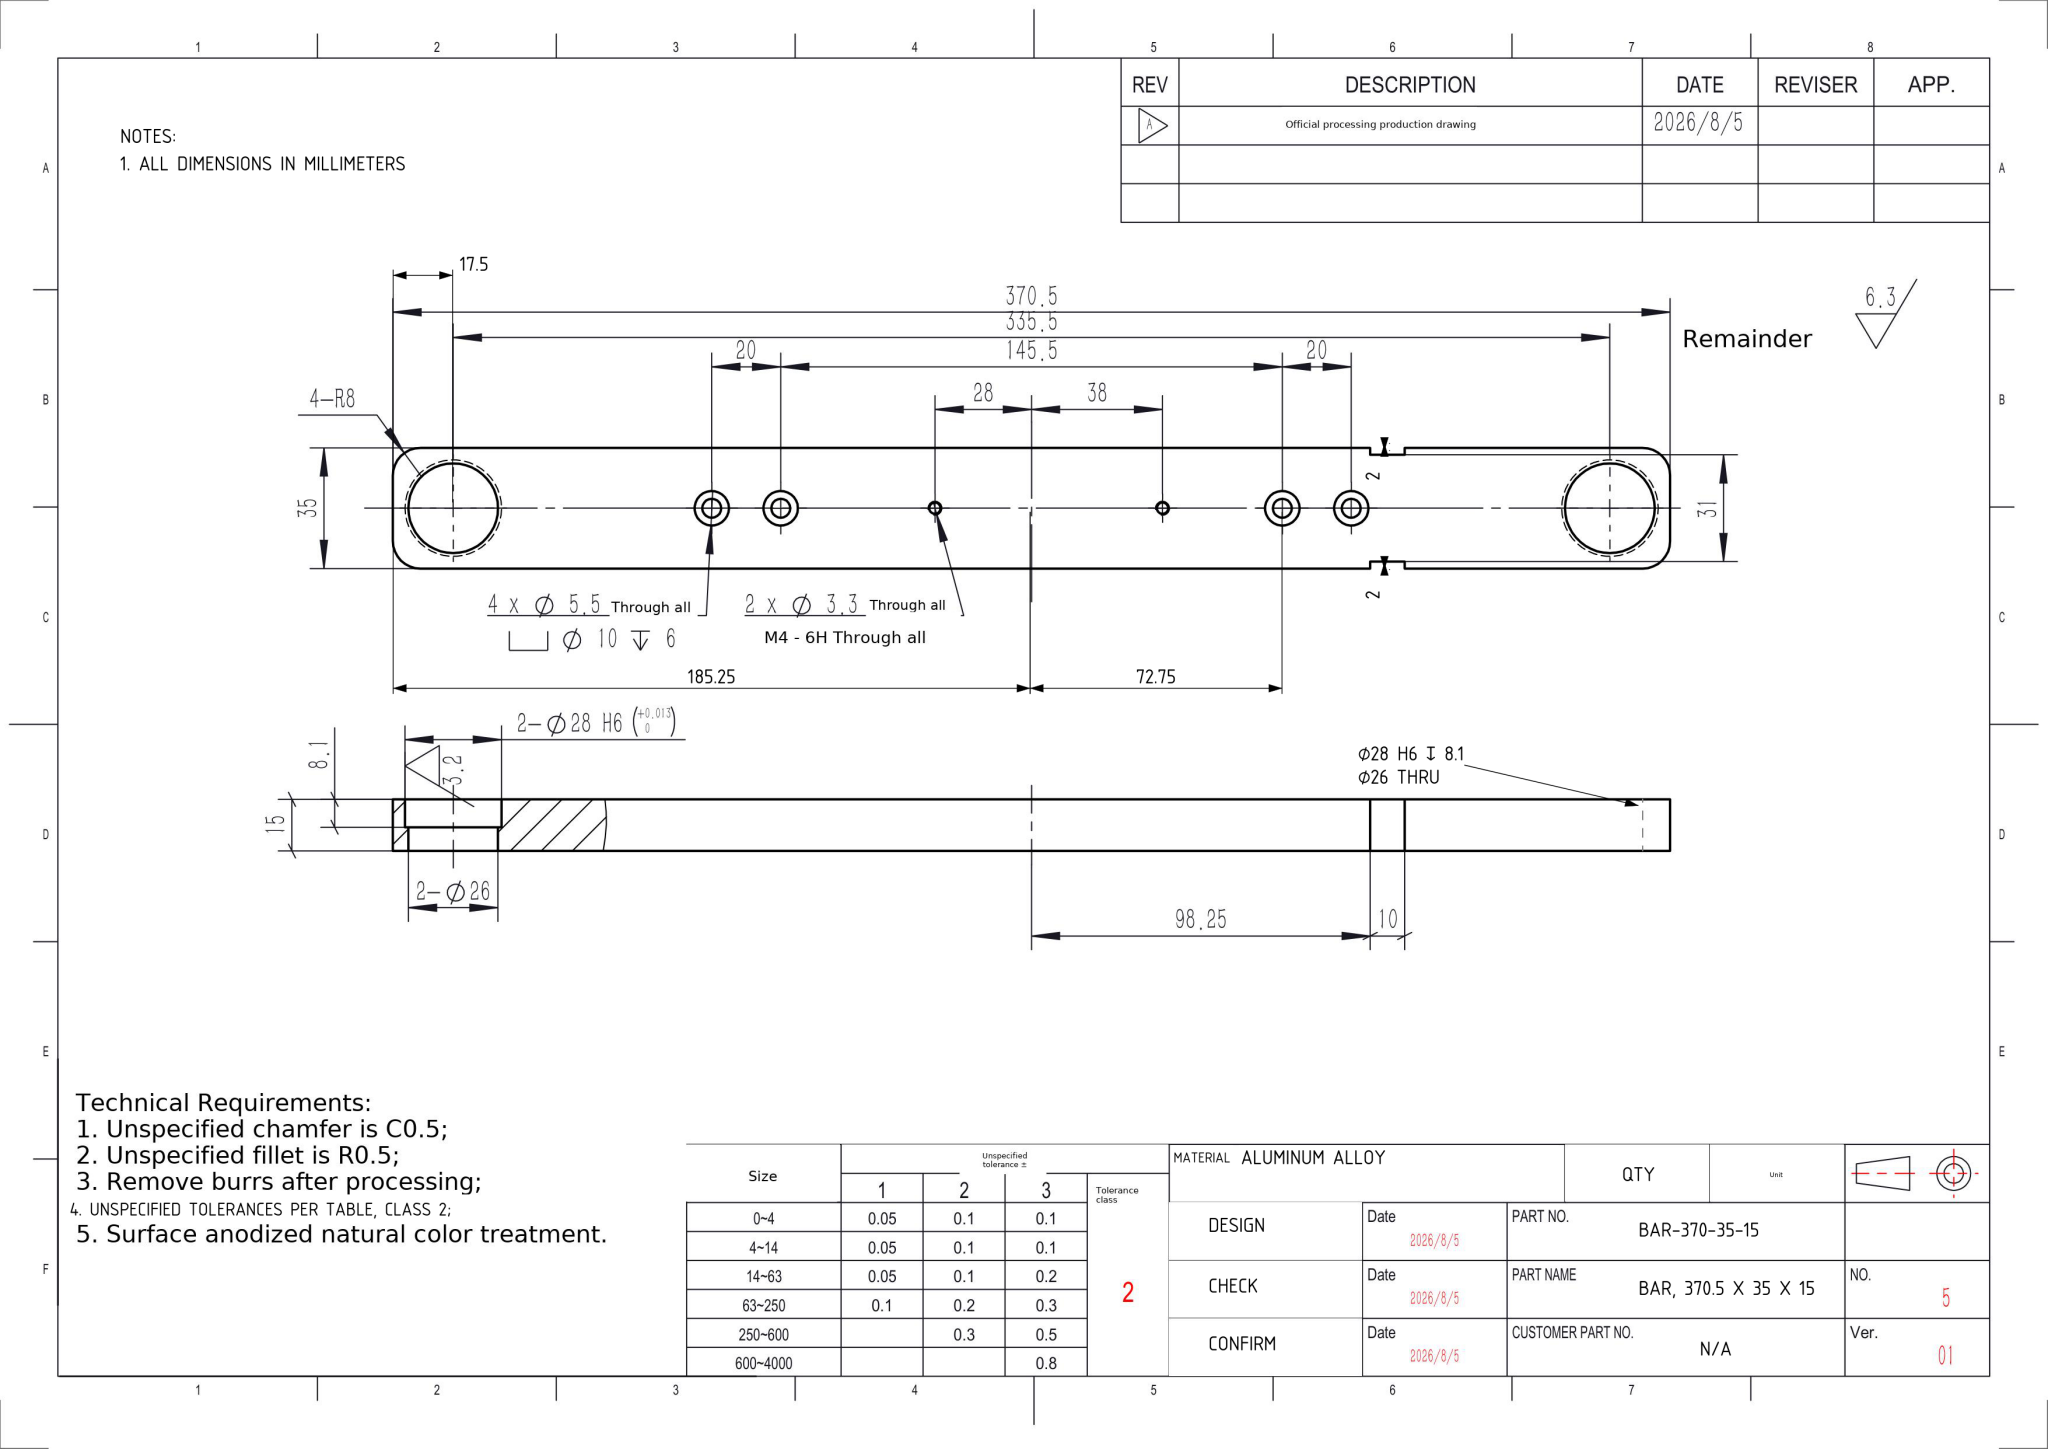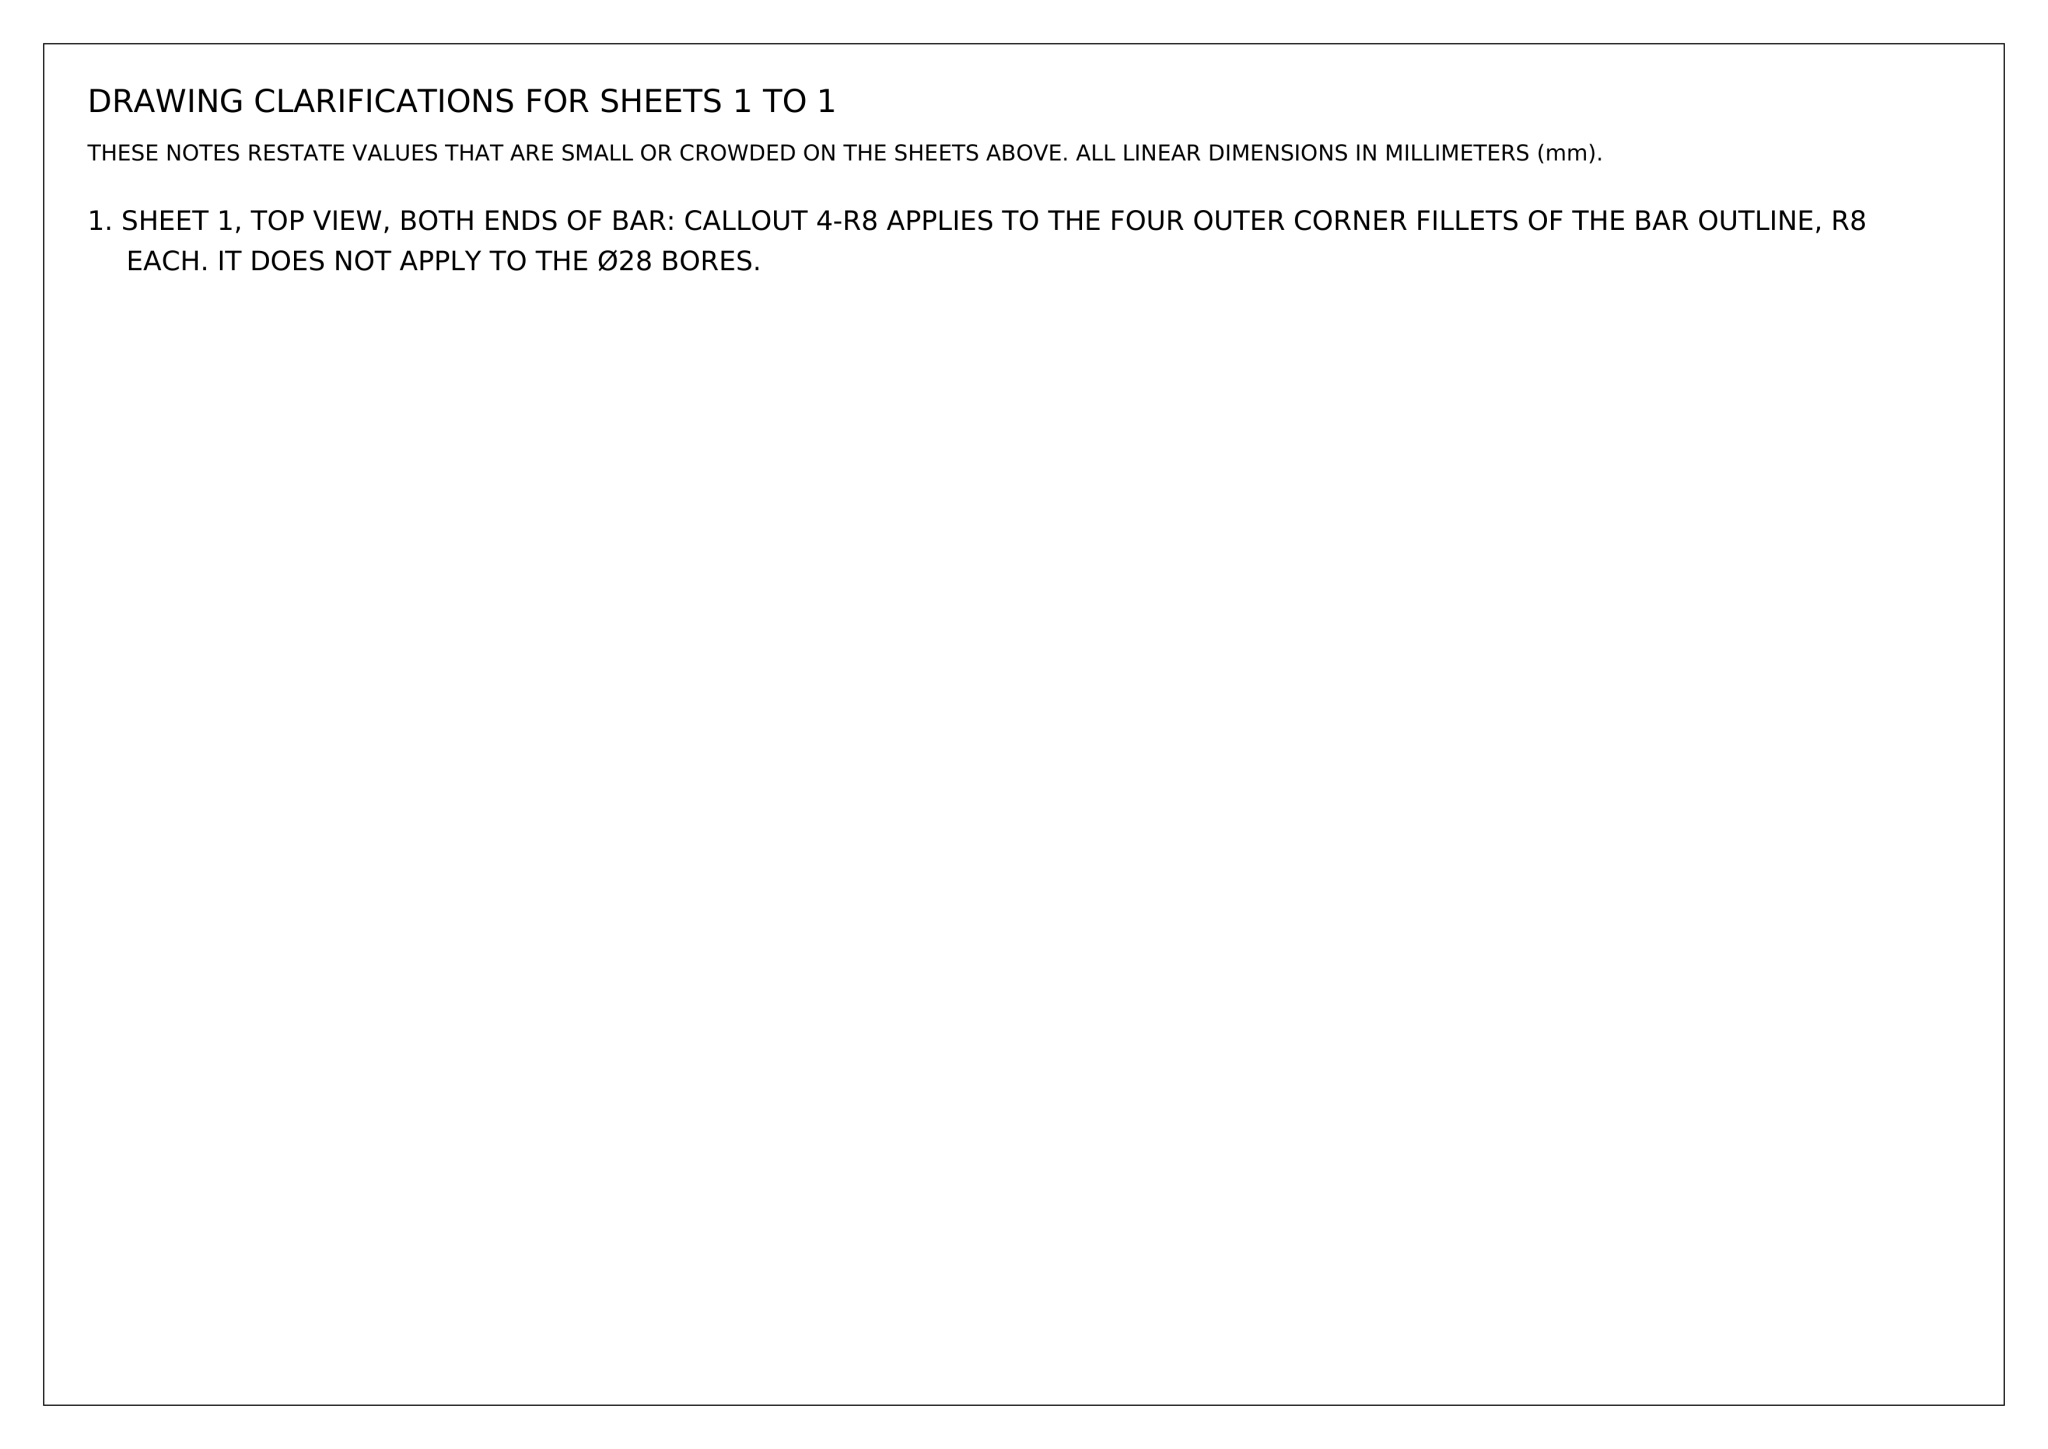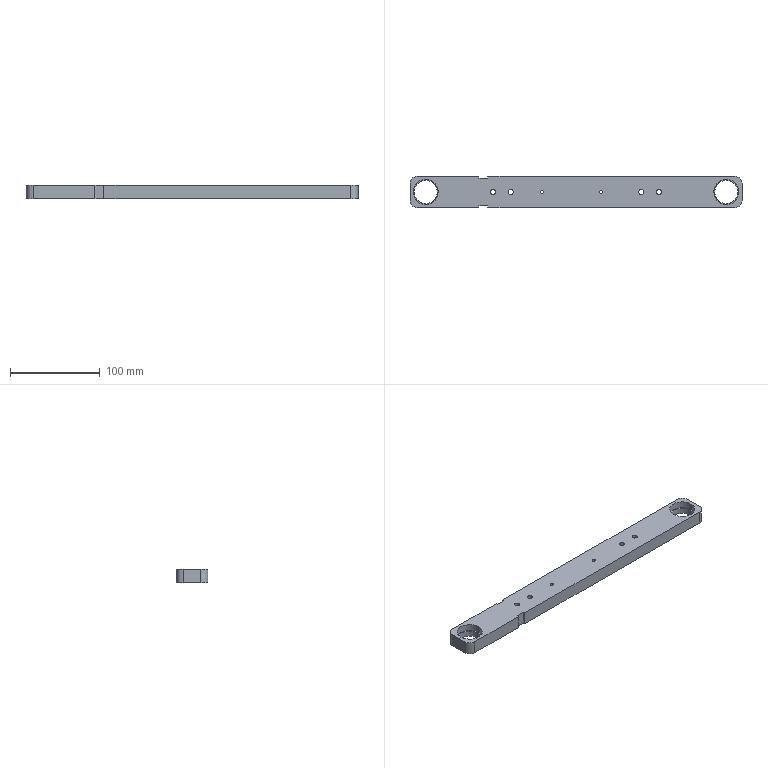Part | NX | mm | 1 solid | 52 faces | box 370.5 x 35 x 15 mm | volume 172790 mm3 | cylinder 32 | plane 20 | commonest cylinder face diameters 10 x8 5.5 x8 26 x4 3.3 x4 28 x4 16 x4